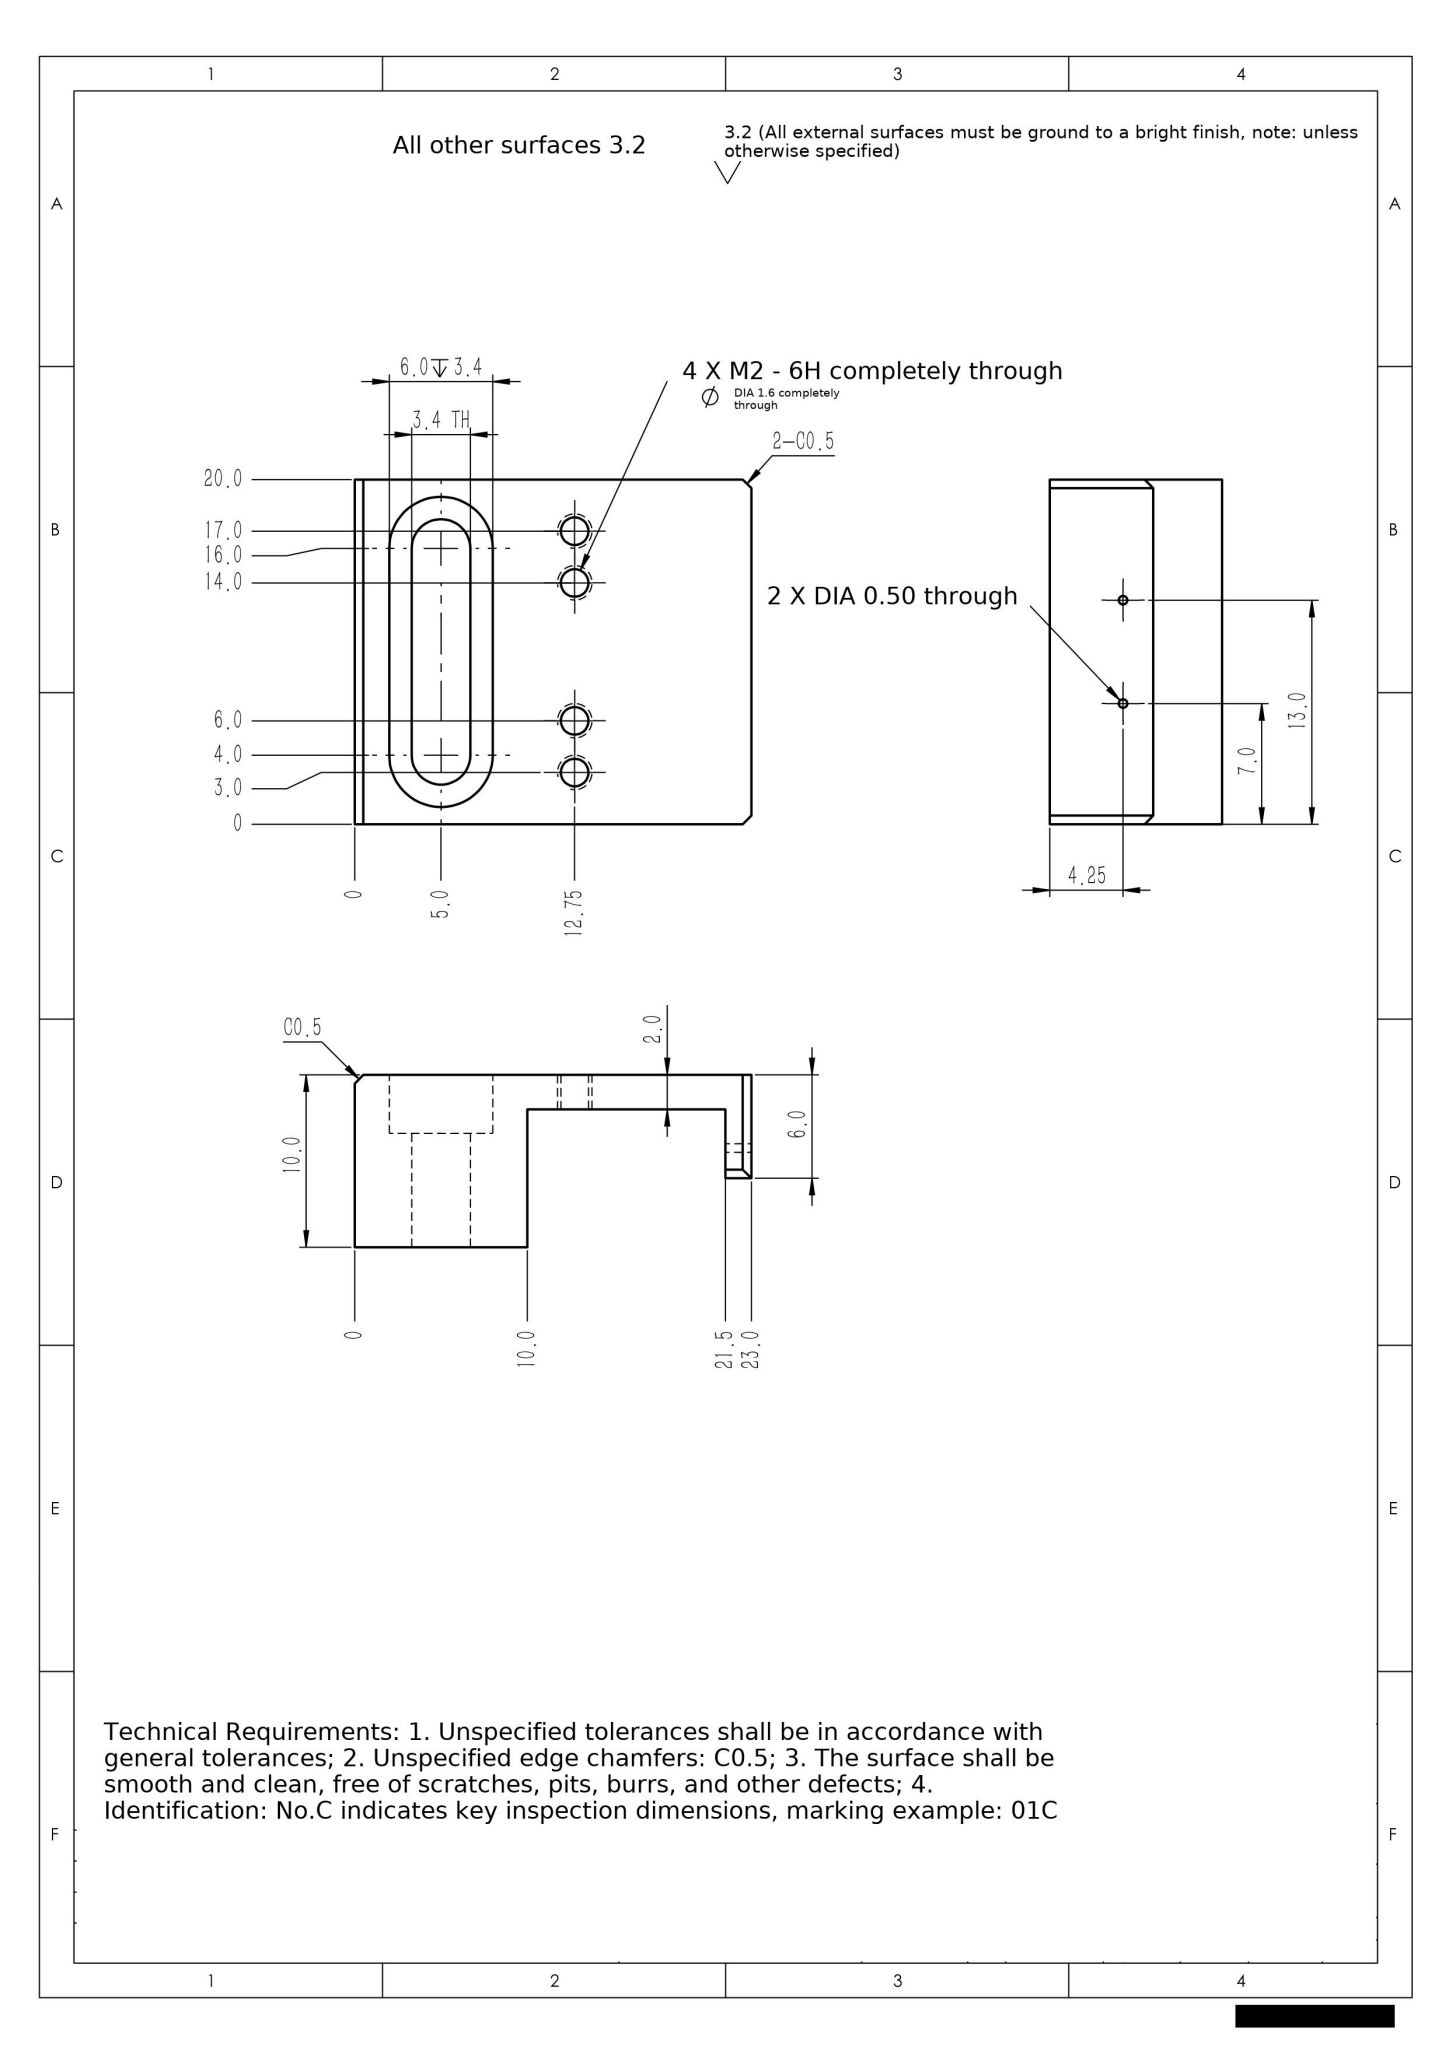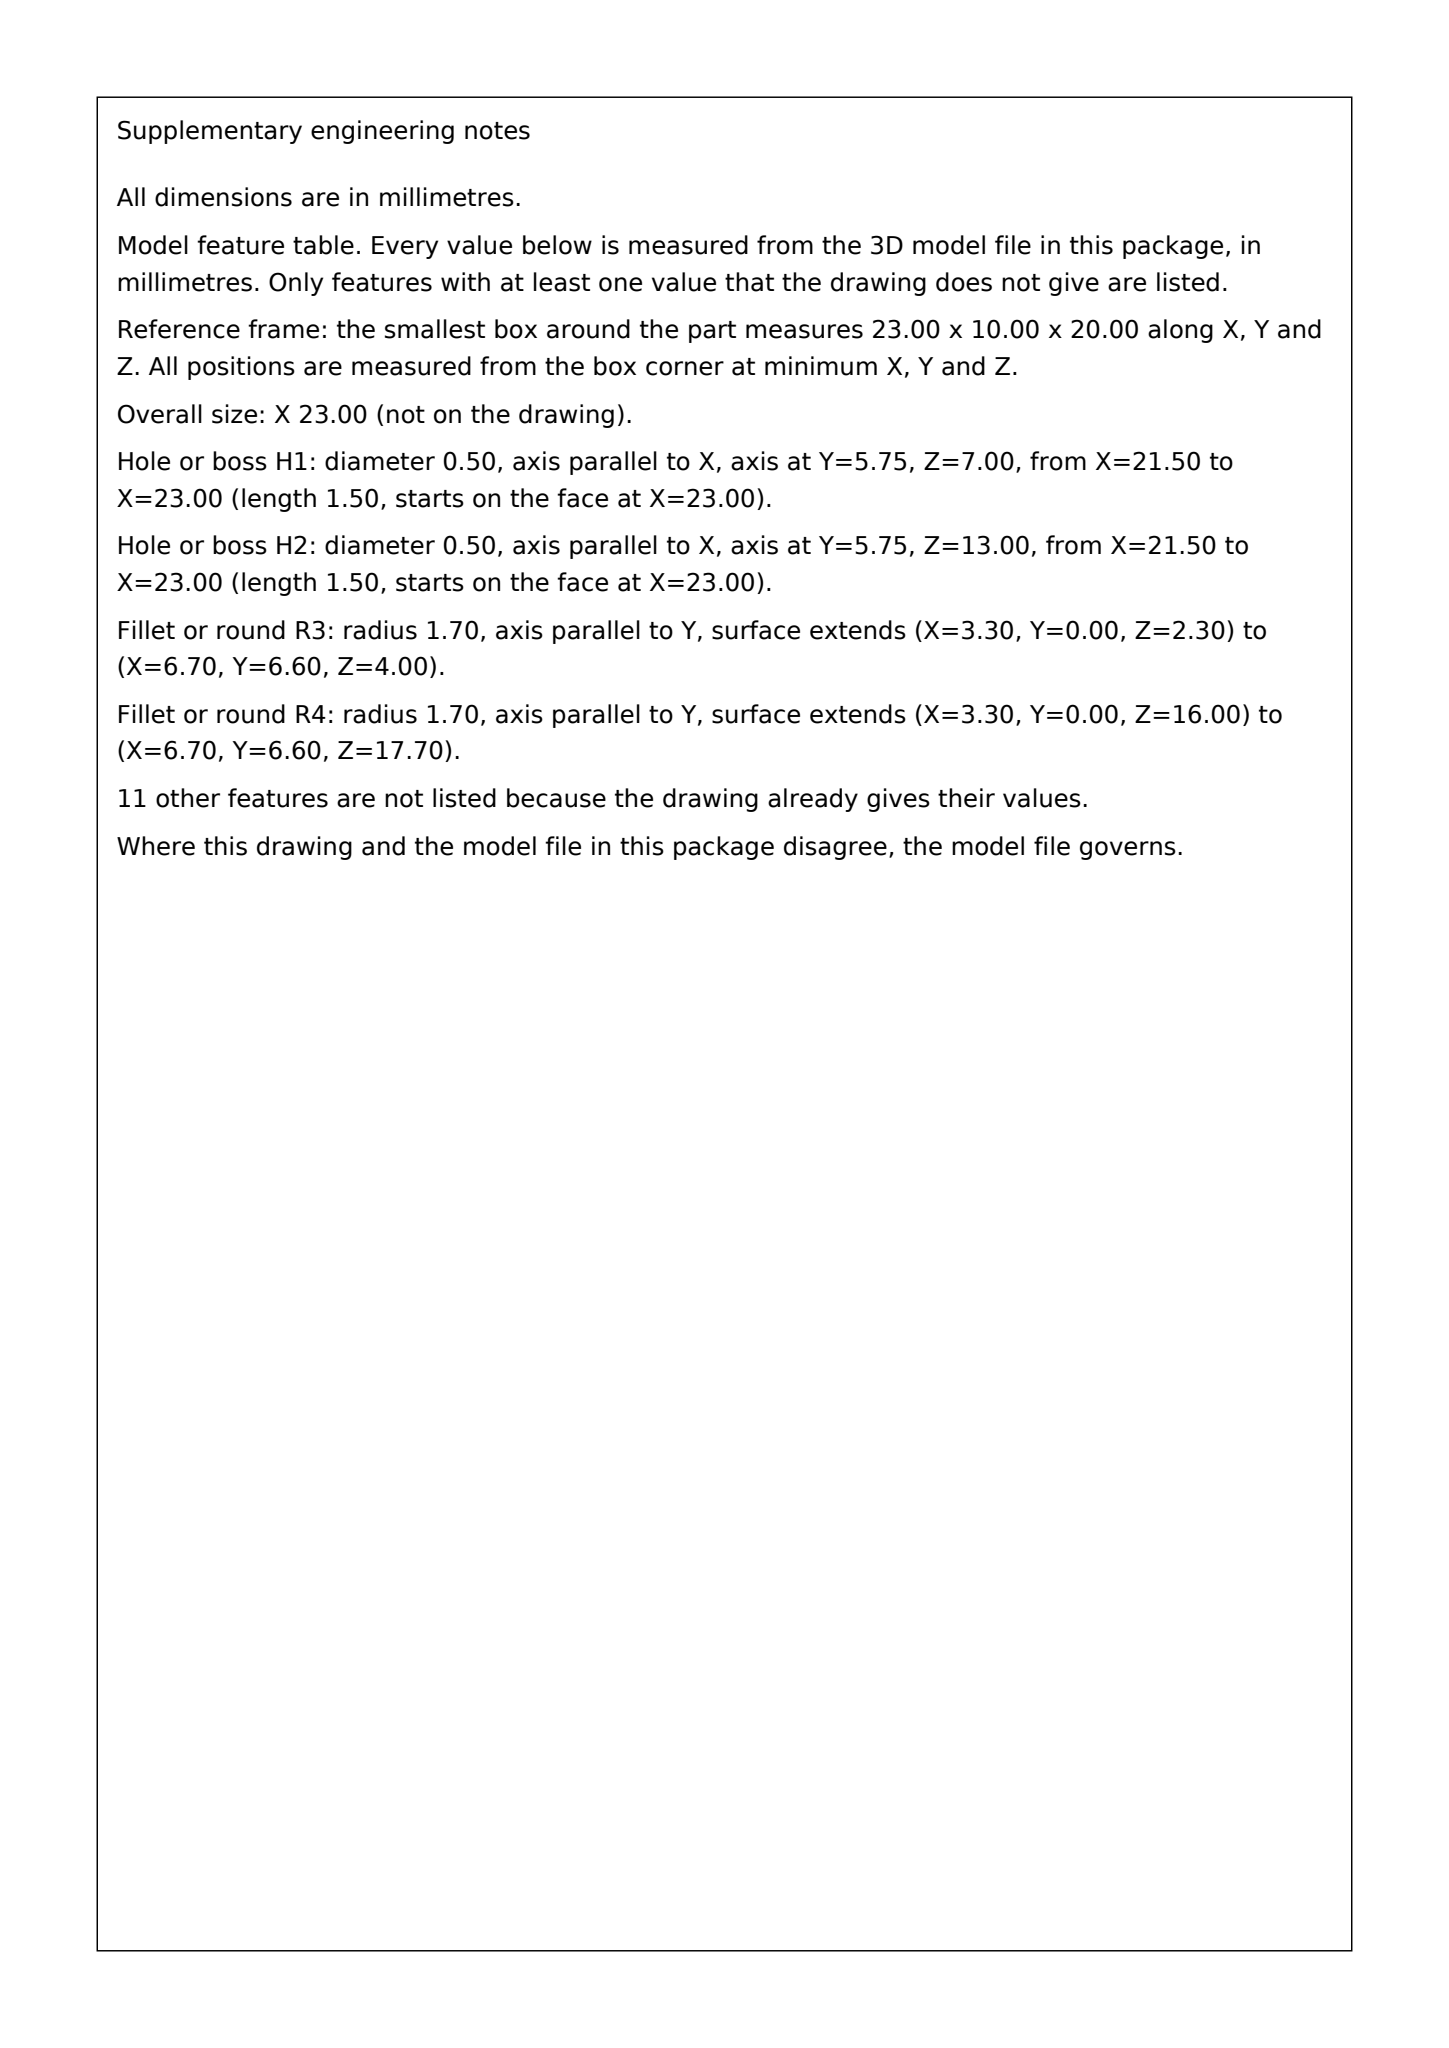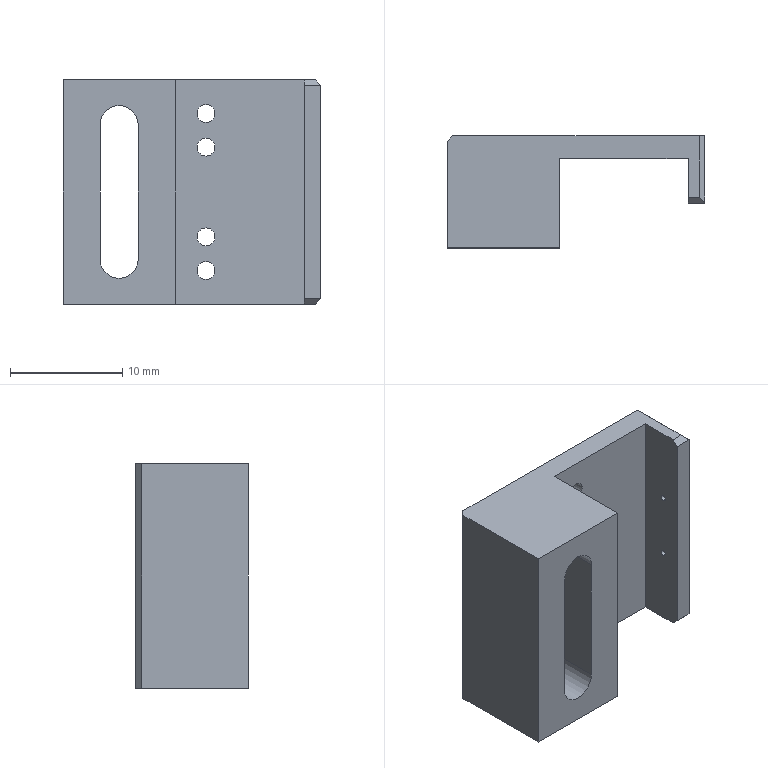Part | SolidWorks | mm | 1 solid | 38 faces | box 23 x 10 x 20 mm | volume 1949 mm3 | plane 20 | cylinder 18 | commonest cylinder face diameters 1.6 x8 0.5 x4 6 x3 3.4 x3